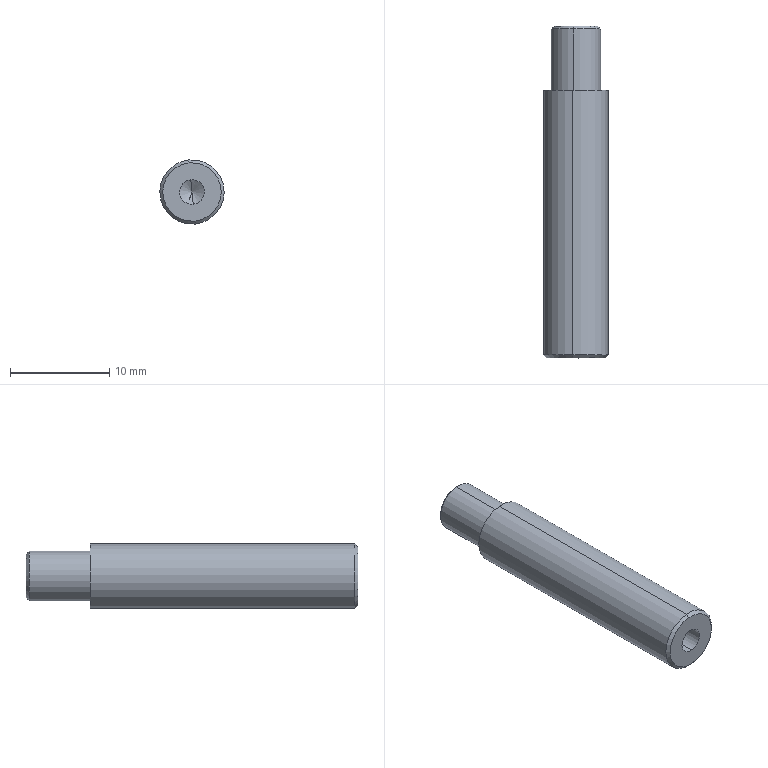Component | SolidWorks | DZ.KX.203-TC1505-30-09-01-05-12-1 | 1 solid | 15 faces | box 6.5 x 33.5 x 6.5 mm | volume 952 mm3 | cone 6 | cylinder 6 | plane 3 | commonest cylinder face diameters 2.5 x2 5 x2 6.5 x2 | material Plain Carbon Steel
build123d program:
from build123d import *

# Parameters (mm, degrees)
SKETCH1_R             = 3.25
BOSS_EXTRUDE1_DEPTH   = 27
SKETCH2_R             = 2.5
BOSS_EXTRUDE2_DEPTH   = 6.5
M3_TAPPED_HOLE1_D     = 2.5
M3_TAPPED_HOLE1_DEPTH = 14
M3_TAPPED_HOLE1_TIP   = 0.7511
CHAMFER1_SIZE         = 0.3


with BuildPart() as part:
    # Sketch1 → Boss-Extrude1 (new body)
    with BuildSketch(Plane(origin=(0, 0, 0), x_dir=(0, 0, -1), z_dir=(1, 0, 0))):
        Circle(SKETCH1_R)
    extrude(amount=BOSS_EXTRUDE1_DEPTH)

    # Sketch2 → Boss-Extrude2 (add)
    with BuildSketch(Plane.ZY):
        with Locations(Location((0, 0, 0), (0, 0, 180))):
            Circle(SKETCH2_R)
    extrude(amount=BOSS_EXTRUDE2_DEPTH)

    # M3 Tapped Hole1
    with Locations(Plane(origin=(27, 0, 0), x_dir=(0, 0, -1), z_dir=(1, 0, 0))):
        with Locations((0, 0)):
            Hole(M3_TAPPED_HOLE1_D / 2, depth=M3_TAPPED_HOLE1_DEPTH)
            with Locations((0, 0, -(M3_TAPPED_HOLE1_DEPTH + M3_TAPPED_HOLE1_TIP / 2))):  # 118° drill point
                Cone(0, M3_TAPPED_HOLE1_D / 2, M3_TAPPED_HOLE1_TIP, mode=Mode.SUBTRACT)

    # Chamfer1
    chamfer1_edges = [part.edges().sort_by_distance(p)[0] for p in [
        (27, 0, 3.25),
        (-6.5, 0, 2.5),
    ]]
    chamfer(chamfer1_edges, length=CHAMFER1_SIZE)


solid = part.part

# Placed as in the assembly
solid = solid.moved(Location((273.5, -525.807, -37.44), (0, 0, -90)))
STEP:
#1=COLOUR_RGB('',0.7922,0.8196,0.9333);
#2=FILL_AREA_STYLE_COLOUR('',#1);
#3=FILL_AREA_STYLE('',(#2));
#4=SURFACE_STYLE_FILL_AREA(#3);
#5=SURFACE_SIDE_STYLE('',(#4));
#6=SURFACE_STYLE_USAGE(.BOTH.,#5);
#7=PRESENTATION_STYLE_ASSIGNMENT((#6));
#8=CARTESIAN_POINT('',(10.759,-20.445,-1.388));
#9=VERTEX_POINT('',#8);
#10=CARTESIAN_POINT('',(10.776,-20.445,-1.56));
#11=VERTEX_POINT('',#10);
#12=CARTESIAN_POINT('',(10.768,-20.445,-1.474));
#13=DIRECTION('',(0.,1.,-0.));
#14=DIRECTION('',(-0.0993,0.,0.9951));
#15=AXIS2_PLACEMENT_3D('',#12,#13,#14);
#16=CIRCLE('',#15,0.08661);
#17=EDGE_CURVE('',#9,#11,#16,.T.);
#18=ORIENTED_EDGE('',*,*,#17,.F.);
#19=CARTESIAN_POINT('',(10.758,-20.457,-1.376));
#20=VERTEX_POINT('',#19);
#21=CARTESIAN_POINT('',(10.759,-20.445,-1.388));
#22=DIRECTION('',(-0.07022,-0.7071,0.7036));
#23=VECTOR('',#22,39.37);
#24=LINE('',#21,#23);
#25=EDGE_CURVE('',#9,#20,#24,.T.);
#26=ORIENTED_EDGE('',*,*,#25,.T.);
#27=CARTESIAN_POINT('',(10.777,-20.457,-1.572));
#28=VERTEX_POINT('',#27);
#29=CARTESIAN_POINT('',(10.768,-20.457,-1.474));
#30=DIRECTION('',(-0.,-1.,0.));
#31=DIRECTION('',(-0.0993,0.,0.9951));
#32=AXIS2_PLACEMENT_3D('',#29,#30,#31);
#33=CIRCLE('',#32,0.09843);
#34=EDGE_CURVE('',#28,#20,#33,.T.);
#35=ORIENTED_EDGE('',*,*,#34,.F.);
#36=CARTESIAN_POINT('',(10.776,-20.445,-1.56));
#37=DIRECTION('',(0.07022,-0.7071,-0.7036));
#38=VECTOR('',#37,39.37);
#39=LINE('',#36,#38);
#40=EDGE_CURVE('',#11,#28,#39,.T.);
#41=ORIENTED_EDGE('',*,*,#40,.F.);
#42=EDGE_LOOP('',(#18,#26,#35,#41));
#43=FACE_OUTER_BOUND('',#42,.T.);
#44=CARTESIAN_POINT('',(10.768,-20.445,-1.474));
#45=DIRECTION('',(-0.,-1.,0.));
#46=DIRECTION('',(0.0993,0.,-0.9951));
#47=AXIS2_PLACEMENT_3D('',#44,#45,#46);
#48=CONICAL_SURFACE('',#47,0.08661,0.7854);
#49=ADVANCED_FACE('',(#43),#48,.T.);
#50=CARTESIAN_POINT('',(10.779,-21.764,-1.59));
#51=VERTEX_POINT('',#50);
#52=CARTESIAN_POINT('',(10.756,-21.764,-1.358));
#53=VERTEX_POINT('',#52);
#54=CARTESIAN_POINT('',(10.768,-21.764,-1.474));
#55=DIRECTION('',(-0.,-1.,0.));
#56=DIRECTION('',(0.0993,0.,-0.9951));
#57=AXIS2_PLACEMENT_3D('',#54,#55,#56);
#58=CIRCLE('',#57,0.1161);
#59=EDGE_CURVE('',#51,#53,#58,.T.);
#60=ORIENTED_EDGE('',*,*,#59,.F.);
#61=CARTESIAN_POINT('',(10.78,-21.752,-1.601));
#62=VERTEX_POINT('',#61);
#63=CARTESIAN_POINT('',(10.779,-21.764,-1.59));
#64=DIRECTION('',(0.07022,0.7071,-0.7036));
#65=VECTOR('',#64,39.37);
#66=LINE('',#63,#65);
#67=EDGE_CURVE('',#51,#62,#66,.T.);
#68=ORIENTED_EDGE('',*,*,#67,.T.);
#69=CARTESIAN_POINT('',(10.755,-21.752,-1.347));
#70=VERTEX_POINT('',#69);
#71=CARTESIAN_POINT('',(10.768,-21.752,-1.474));
#72=DIRECTION('',(0.,1.,-0.));
#73=DIRECTION('',(0.0993,0.,-0.9951));
#74=AXIS2_PLACEMENT_3D('',#71,#72,#73);
#75=CIRCLE('',#74,0.128);
#76=EDGE_CURVE('',#70,#62,#75,.T.);
#77=ORIENTED_EDGE('',*,*,#76,.F.);
#78=CARTESIAN_POINT('',(10.756,-21.764,-1.358));
#79=DIRECTION('',(-0.07022,0.7071,0.7036));
#80=VECTOR('',#79,39.37);
#81=LINE('',#78,#80);
#82=EDGE_CURVE('',#53,#70,#81,.T.);
#83=ORIENTED_EDGE('',*,*,#82,.F.);
#84=EDGE_LOOP('',(#60,#68,#77,#83));
#85=FACE_OUTER_BOUND('',#84,.T.);
#86=CARTESIAN_POINT('',(10.768,-21.764,-1.474));
#87=DIRECTION('',(0.,1.,-0.));
#88=DIRECTION('',(-0.0993,0.,0.9951));
#89=AXIS2_PLACEMENT_3D('',#86,#87,#88);
#90=CONICAL_SURFACE('',#89,0.1161,0.7854);
#91=ADVANCED_FACE('',(#85),#90,.T.);
#92=CARTESIAN_POINT('',(10.763,-21.213,-1.425));
#93=VERTEX_POINT('',#92);
#94=CARTESIAN_POINT('',(10.773,-21.213,-1.523));
#95=VERTEX_POINT('',#94);
#96=CARTESIAN_POINT('',(10.768,-21.213,-1.474));
#97=DIRECTION('',(-0.,-1.,0.));
#98=DIRECTION('',(0.0993,0.,-0.9951));
#99=AXIS2_PLACEMENT_3D('',#96,#97,#98);
#100=CIRCLE('',#99,0.04921);
#101=EDGE_CURVE('',#93,#95,#100,.T.);
#102=ORIENTED_EDGE('',*,*,#101,.F.);
#103=CARTESIAN_POINT('',(10.763,-21.764,-1.425));
#104=VERTEX_POINT('',#103);
#105=CARTESIAN_POINT('',(10.763,-21.764,-1.425));
#106=DIRECTION('',(-0.,-1.,0.));
#107=VECTOR('',#106,39.37);
#108=LINE('',#105,#107);
#109=EDGE_CURVE('',#93,#104,#108,.T.);
#110=ORIENTED_EDGE('',*,*,#109,.T.);
#111=CARTESIAN_POINT('',(10.773,-21.764,-1.523));
#112=VERTEX_POINT('',#111);
#113=CARTESIAN_POINT('',(10.768,-21.764,-1.474));
#114=DIRECTION('',(-0.,-1.,0.));
#115=DIRECTION('',(0.0993,0.,-0.9951));
#116=AXIS2_PLACEMENT_3D('',#113,#114,#115);
#117=CIRCLE('',#116,0.04921);
#118=EDGE_CURVE('',#104,#112,#117,.T.);
#119=ORIENTED_EDGE('',*,*,#118,.T.);
#120=CARTESIAN_POINT('',(10.773,-21.764,-1.523));
#121=DIRECTION('',(-0.,-1.,0.));
#122=VECTOR('',#121,39.37);
#123=LINE('',#120,#122);
#124=EDGE_CURVE('',#95,#112,#123,.T.);
#125=ORIENTED_EDGE('',*,*,#124,.F.);
#126=EDGE_LOOP('',(#102,#110,#119,#125));
#127=FACE_OUTER_BOUND('',#126,.T.);
#128=CARTESIAN_POINT('',(10.768,-21.764,-1.474));
#129=DIRECTION('',(-0.,-1.,0.));
#130=DIRECTION('',(0.0993,0.,-0.9951));
#131=AXIS2_PLACEMENT_3D('',#128,#129,#130);
#132=CYLINDRICAL_SURFACE('',#131,0.04921);
#133=ADVANCED_FACE('',(#127),#132,.F.);
#134=CARTESIAN_POINT('',(10.768,-21.183,-1.474));
#135=VERTEX_POINT('',#134);
#136=CARTESIAN_POINT('',(10.773,-21.213,-1.523));
#137=DIRECTION('',(0.08512,-0.515,-0.8529));
#138=VECTOR('',#137,39.37);
#139=LINE('',#136,#138);
#140=EDGE_CURVE('',#135,#95,#139,.T.);
#141=ORIENTED_EDGE('',*,*,#140,.F.);
#142=CARTESIAN_POINT('',(10.763,-21.213,-1.425));
#143=DIRECTION('',(-0.08512,-0.515,0.8529));
#144=VECTOR('',#143,39.37);
#145=LINE('',#142,#144);
#146=EDGE_CURVE('',#135,#93,#145,.T.);
#147=ORIENTED_EDGE('',*,*,#146,.T.);
#148=ORIENTED_EDGE('',*,*,#101,.T.);
#149=EDGE_LOOP('',(#141,#147,#148));
#150=FACE_OUTER_BOUND('',#149,.T.);
#151=CARTESIAN_POINT('',(10.768,-21.213,-1.474));
#152=DIRECTION('',(-0.,-1.,0.));
#153=DIRECTION('',(0.0993,0.,-0.9951));
#154=AXIS2_PLACEMENT_3D('',#151,#152,#153);
#155=CONICAL_SURFACE('',#154,0.04921,1.03);
#156=ADVANCED_FACE('',(#150),#155,.F.);
#157=ORIENTED_EDGE('',*,*,#34,.T.);
#158=CARTESIAN_POINT('',(10.758,-20.701,-1.376));
#159=VERTEX_POINT('',#158);
#160=CARTESIAN_POINT('',(10.758,-20.445,-1.376));
#161=DIRECTION('',(-0.,-1.,0.));
#162=VECTOR('',#161,39.37);
#163=LINE('',#160,#162);
#164=EDGE_CURVE('',#20,#159,#163,.T.);
#165=ORIENTED_EDGE('',*,*,#164,.T.);
#166=CARTESIAN_POINT('',(10.777,-20.701,-1.572));
#167=VERTEX_POINT('',#166);
#168=CARTESIAN_POINT('',(10.768,-20.701,-1.474));
#169=DIRECTION('',(0.,1.,-0.));
#170=DIRECTION('',(0.0993,0.,-0.9951));
#171=AXIS2_PLACEMENT_3D('',#168,#169,#170);
#172=CIRCLE('',#171,0.09843);
#173=EDGE_CURVE('',#159,#167,#172,.T.);
#174=ORIENTED_EDGE('',*,*,#173,.T.);
#175=CARTESIAN_POINT('',(10.777,-20.445,-1.572));
#176=DIRECTION('',(-0.,-1.,0.));
#177=VECTOR('',#176,39.37);
#178=LINE('',#175,#177);
#179=EDGE_CURVE('',#28,#167,#178,.T.);
#180=ORIENTED_EDGE('',*,*,#179,.F.);
#181=EDGE_LOOP('',(#157,#165,#174,#180));
#182=FACE_OUTER_BOUND('',#181,.T.);
#183=CARTESIAN_POINT('',(10.768,-20.445,-1.474));
#184=DIRECTION('',(-0.,-1.,0.));
#185=DIRECTION('',(0.0993,0.,-0.9951));
#186=AXIS2_PLACEMENT_3D('',#183,#184,#185);
#187=CYLINDRICAL_SURFACE('',#186,0.09843);
#188=ADVANCED_FACE('',(#182),#187,.T.);
#189=ORIENTED_EDGE('',*,*,#76,.T.);
#190=CARTESIAN_POINT('',(10.78,-20.701,-1.601));
#191=VERTEX_POINT('',#190);
#192=CARTESIAN_POINT('',(10.78,-21.764,-1.601));
#193=DIRECTION('',(0.,1.,-0.));
#194=VECTOR('',#193,39.37);
#195=LINE('',#192,#194);
#196=EDGE_CURVE('',#62,#191,#195,.T.);
#197=ORIENTED_EDGE('',*,*,#196,.T.);
#198=CARTESIAN_POINT('',(10.755,-20.701,-1.347));
#199=VERTEX_POINT('',#198);
#200=CARTESIAN_POINT('',(10.768,-20.701,-1.474));
#201=DIRECTION('',(-0.,-1.,0.));
#202=DIRECTION('',(0.0993,0.,-0.9951));
#203=AXIS2_PLACEMENT_3D('',#200,#201,#202);
#204=CIRCLE('',#203,0.128);
#205=EDGE_CURVE('',#191,#199,#204,.T.);
#206=ORIENTED_EDGE('',*,*,#205,.T.);
#207=CARTESIAN_POINT('',(10.755,-21.764,-1.347));
#208=DIRECTION('',(0.,1.,-0.));
#209=VECTOR('',#208,39.37);
#210=LINE('',#207,#209);
#211=EDGE_CURVE('',#70,#199,#210,.T.);
#212=ORIENTED_EDGE('',*,*,#211,.F.);
#213=EDGE_LOOP('',(#189,#197,#206,#212));
#214=FACE_OUTER_BOUND('',#213,.T.);
#215=CARTESIAN_POINT('',(10.768,-21.764,-1.474));
#216=DIRECTION('',(0.,1.,-0.));
#217=DIRECTION('',(-0.0993,0.,0.9951));
#218=AXIS2_PLACEMENT_3D('',#215,#216,#217);
#219=CYLINDRICAL_SURFACE('',#218,0.128);
#220=ADVANCED_FACE('',(#214),#219,.T.);
#221=CARTESIAN_POINT('',(10.768,-20.701,-1.474));
#222=DIRECTION('',(-0.,-1.,0.));
#223=DIRECTION('',(0.0993,0.,-0.9951));
#224=AXIS2_PLACEMENT_3D('',#221,#222,#223);
#225=CIRCLE('',#224,0.128);
#226=EDGE_CURVE('',#199,#191,#225,.T.);
#227=ORIENTED_EDGE('',*,*,#226,.F.);
#228=ORIENTED_EDGE('',*,*,#205,.F.);
#229=EDGE_LOOP('',(#227,#228));
#230=FACE_OUTER_BOUND('',#229,.T.);
#231=CARTESIAN_POINT('',(10.768,-20.701,-1.474));
#232=DIRECTION('',(0.,1.,-0.));
#233=DIRECTION('',(0.0993,0.,-0.9951));
#234=AXIS2_PLACEMENT_3D('',#231,#232,#233);
#235=CIRCLE('',#234,0.09843);
#236=EDGE_CURVE('',#167,#159,#235,.T.);
#237=ORIENTED_EDGE('',*,*,#236,.F.);
#238=ORIENTED_EDGE('',*,*,#173,.F.);
#239=EDGE_LOOP('',(#237,#238));
#240=FACE_BOUND('',#239,.T.);
#241=CARTESIAN_POINT('',(10.768,-20.701,-1.474));
#242=DIRECTION('',(-0.,-1.,0.));
#243=DIRECTION('',(0.0993,-0.,-0.9951));
#244=AXIS2_PLACEMENT_3D('',#241,#242,#243);
#245=PLANE('',#244);
#246=ADVANCED_FACE('',(#230,#240),#245,.F.);
#247=ORIENTED_EDGE('',*,*,#196,.F.);
#248=CARTESIAN_POINT('',(10.768,-21.752,-1.474));
#249=DIRECTION('',(0.,1.,-0.));
#250=DIRECTION('',(0.0993,0.,-0.9951));
#251=AXIS2_PLACEMENT_3D('',#248,#249,#250);
#252=CIRCLE('',#251,0.128);
#253=EDGE_CURVE('',#62,#70,#252,.T.);
#254=ORIENTED_EDGE('',*,*,#253,.T.);
#255=ORIENTED_EDGE('',*,*,#211,.T.);
#256=ORIENTED_EDGE('',*,*,#226,.T.);
#257=EDGE_LOOP('',(#247,#254,#255,#256));
#258=FACE_OUTER_BOUND('',#257,.T.);
#259=CARTESIAN_POINT('',(10.768,-21.764,-1.474));
#260=DIRECTION('',(0.,1.,-0.));
#261=DIRECTION('',(-0.0993,0.,0.9951));
#262=AXIS2_PLACEMENT_3D('',#259,#260,#261);
#263=CYLINDRICAL_SURFACE('',#262,0.128);
#264=ADVANCED_FACE('',(#258),#263,.T.);
#265=CARTESIAN_POINT('',(10.768,-21.764,-1.474));
#266=DIRECTION('',(-0.,-1.,0.));
#267=DIRECTION('',(0.0993,0.,-0.9951));
#268=AXIS2_PLACEMENT_3D('',#265,#266,#267);
#269=CIRCLE('',#268,0.1161);
#270=EDGE_CURVE('',#53,#51,#269,.T.);
#271=ORIENTED_EDGE('',*,*,#270,.T.);
#272=ORIENTED_EDGE('',*,*,#59,.T.);
#273=EDGE_LOOP('',(#271,#272));
#274=FACE_OUTER_BOUND('',#273,.T.);
#275=CARTESIAN_POINT('',(10.768,-21.764,-1.474));
#276=DIRECTION('',(-0.,-1.,0.));
#277=DIRECTION('',(0.0993,0.,-0.9951));
#278=AXIS2_PLACEMENT_3D('',#275,#276,#277);
#279=CIRCLE('',#278,0.04921);
#280=EDGE_CURVE('',#112,#104,#279,.T.);
#281=ORIENTED_EDGE('',*,*,#280,.F.);
#282=ORIENTED_EDGE('',*,*,#118,.F.);
#283=EDGE_LOOP('',(#281,#282));
#284=FACE_BOUND('',#283,.T.);
#285=CARTESIAN_POINT('',(10.768,-21.764,-1.474));
#286=DIRECTION('',(-0.,-1.,0.));
#287=DIRECTION('',(0.0993,-0.,-0.9951));
#288=AXIS2_PLACEMENT_3D('',#285,#286,#287);
#289=PLANE('',#288);
#290=ADVANCED_FACE('',(#274,#284),#289,.T.);
#291=ORIENTED_EDGE('',*,*,#164,.F.);
#292=CARTESIAN_POINT('',(10.768,-20.457,-1.474));
#293=DIRECTION('',(-0.,-1.,0.));
#294=DIRECTION('',(-0.0993,0.,0.9951));
#295=AXIS2_PLACEMENT_3D('',#292,#293,#294);
#296=CIRCLE('',#295,0.09843);
#297=EDGE_CURVE('',#20,#28,#296,.T.);
#298=ORIENTED_EDGE('',*,*,#297,.T.);
#299=ORIENTED_EDGE('',*,*,#179,.T.);
#300=ORIENTED_EDGE('',*,*,#236,.T.);
#301=EDGE_LOOP('',(#291,#298,#299,#300));
#302=FACE_OUTER_BOUND('',#301,.T.);
#303=CARTESIAN_POINT('',(10.768,-20.445,-1.474));
#304=DIRECTION('',(-0.,-1.,0.));
#305=DIRECTION('',(0.0993,0.,-0.9951));
#306=AXIS2_PLACEMENT_3D('',#303,#304,#305);
#307=CYLINDRICAL_SURFACE('',#306,0.09843);
#308=ADVANCED_FACE('',(#302),#307,.T.);
#309=CARTESIAN_POINT('',(10.768,-20.445,-1.474));
#310=DIRECTION('',(0.,1.,-0.));
#311=DIRECTION('',(-0.0993,0.,0.9951));
#312=AXIS2_PLACEMENT_3D('',#309,#310,#311);
#313=CIRCLE('',#312,0.08661);
#314=EDGE_CURVE('',#11,#9,#313,.T.);
#315=ORIENTED_EDGE('',*,*,#314,.T.);
#316=ORIENTED_EDGE('',*,*,#17,.T.);
#317=EDGE_LOOP('',(#315,#316));
#318=FACE_OUTER_BOUND('',#317,.T.);
#319=CARTESIAN_POINT('',(10.768,-20.445,-1.474));
#320=DIRECTION('',(0.,1.,-0.));
#321=DIRECTION('',(-0.0993,0.,0.9951));
#322=AXIS2_PLACEMENT_3D('',#319,#320,#321);
#323=PLANE('',#322);
#324=ADVANCED_FACE('',(#318),#323,.T.);
#325=ORIENTED_EDGE('',*,*,#146,.F.);
#326=ORIENTED_EDGE('',*,*,#140,.T.);
#327=CARTESIAN_POINT('',(10.768,-21.213,-1.474));
#328=DIRECTION('',(-0.,-1.,0.));
#329=DIRECTION('',(0.0993,0.,-0.9951));
#330=AXIS2_PLACEMENT_3D('',#327,#328,#329);
#331=CIRCLE('',#330,0.04921);
#332=EDGE_CURVE('',#95,#93,#331,.T.);
#333=ORIENTED_EDGE('',*,*,#332,.T.);
#334=EDGE_LOOP('',(#325,#326,#333));
#335=FACE_OUTER_BOUND('',#334,.T.);
#336=CARTESIAN_POINT('',(10.768,-21.213,-1.474));
#337=DIRECTION('',(-0.,-1.,0.));
#338=DIRECTION('',(0.0993,0.,-0.9951));
#339=AXIS2_PLACEMENT_3D('',#336,#337,#338);
#340=CONICAL_SURFACE('',#339,0.04921,1.03);
#341=ADVANCED_FACE('',(#335),#340,.F.);
#342=ORIENTED_EDGE('',*,*,#109,.F.);
#343=ORIENTED_EDGE('',*,*,#332,.F.);
#344=ORIENTED_EDGE('',*,*,#124,.T.);
#345=ORIENTED_EDGE('',*,*,#280,.T.);
#346=EDGE_LOOP('',(#342,#343,#344,#345));
#347=FACE_OUTER_BOUND('',#346,.T.);
#348=CARTESIAN_POINT('',(10.768,-21.764,-1.474));
#349=DIRECTION('',(-0.,-1.,0.));
#350=DIRECTION('',(0.0993,0.,-0.9951));
#351=AXIS2_PLACEMENT_3D('',#348,#349,#350);
#352=CYLINDRICAL_SURFACE('',#351,0.04921);
#353=ADVANCED_FACE('',(#347),#352,.F.);
#354=ORIENTED_EDGE('',*,*,#67,.F.);
#355=ORIENTED_EDGE('',*,*,#270,.F.);
#356=ORIENTED_EDGE('',*,*,#82,.T.);
#357=ORIENTED_EDGE('',*,*,#253,.F.);
#358=EDGE_LOOP('',(#354,#355,#356,#357));
#359=FACE_OUTER_BOUND('',#358,.T.);
#360=CARTESIAN_POINT('',(10.768,-21.764,-1.474));
#361=DIRECTION('',(0.,1.,-0.));
#362=DIRECTION('',(-0.0993,0.,0.9951));
#363=AXIS2_PLACEMENT_3D('',#360,#361,#362);
#364=CONICAL_SURFACE('',#363,0.1161,0.7854);
#365=ADVANCED_FACE('',(#359),#364,.T.);
#366=ORIENTED_EDGE('',*,*,#25,.F.);
#367=ORIENTED_EDGE('',*,*,#314,.F.);
#368=ORIENTED_EDGE('',*,*,#40,.T.);
#369=ORIENTED_EDGE('',*,*,#297,.F.);
#370=EDGE_LOOP('',(#366,#367,#368,#369));
#371=FACE_OUTER_BOUND('',#370,.T.);
#372=CARTESIAN_POINT('',(10.768,-20.445,-1.474));
#373=DIRECTION('',(-0.,-1.,0.));
#374=DIRECTION('',(0.0993,0.,-0.9951));
#375=AXIS2_PLACEMENT_3D('',#372,#373,#374);
#376=CONICAL_SURFACE('',#375,0.08661,0.7854);
#377=ADVANCED_FACE('',(#371),#376,.T.);
#378=CLOSED_SHELL('',(#49,#91,#133,#156,#188,#220,#246,#264,#290,#308,#324,#341,#353,#365,#377));
#379=MANIFOLD_SOLID_BREP('',#378);
#380=STYLED_ITEM('',(#7),#379);
#381=(LENGTH_UNIT()NAMED_UNIT(*)SI_UNIT($,.METRE.));
#382=LENGTH_MEASURE_WITH_UNIT(LENGTH_MEASURE(0.0254),#381);
#383=DIMENSIONAL_EXPONENTS(1.,0.,0.,0.,0.,0.,0.);
#384=(CONVERSION_BASED_UNIT('',#382)LENGTH_UNIT()NAMED_UNIT(#383));
#385=UNCERTAINTY_MEASURE_WITH_UNIT(LENGTH_MEASURE(0.00001),#384,'','');
#386=(NAMED_UNIT(*)PLANE_ANGLE_UNIT()SI_UNIT($,.RADIAN.));
#387=(NAMED_UNIT(*)SI_UNIT($,.STERADIAN.)SOLID_ANGLE_UNIT());
#388=(GEOMETRIC_REPRESENTATION_CONTEXT(3)GLOBAL_UNCERTAINTY_ASSIGNED_CONTEXT((#385))GLOBAL_UNIT_ASSIGNED_CONTEXT((#384,#386,#387))REPRESENTATION_CONTEXT('',''));
#389=MECHANICAL_DESIGN_GEOMETRIC_PRESENTATION_REPRESENTATION('',(#380),#388);
#390=PRESENTATION_LAYER_ASSIGNMENT('','',(#380));
#391=CARTESIAN_POINT('',(0.,0.,0.));
#392=DIRECTION('',(0.,0.,1.));
#393=DIRECTION('',(1.,0.,0.));
#394=AXIS2_PLACEMENT_3D('',#391,#392,#393);
#395=(LENGTH_UNIT()NAMED_UNIT(*)SI_UNIT($,.METRE.));
#396=LENGTH_MEASURE_WITH_UNIT(LENGTH_MEASURE(0.0254),#395);
#397=DIMENSIONAL_EXPONENTS(1.,0.,0.,0.,0.,0.,0.);
#398=(CONVERSION_BASED_UNIT('',#396)LENGTH_UNIT()NAMED_UNIT(#397));
#399=UNCERTAINTY_MEASURE_WITH_UNIT(LENGTH_MEASURE(0.00001),#398,'','');
#400=(NAMED_UNIT(*)PLANE_ANGLE_UNIT()SI_UNIT($,.RADIAN.));
#401=(NAMED_UNIT(*)SI_UNIT($,.STERADIAN.)SOLID_ANGLE_UNIT());
#402=(GEOMETRIC_REPRESENTATION_CONTEXT(3)GLOBAL_UNCERTAINTY_ASSIGNED_CONTEXT((#399))GLOBAL_UNIT_ASSIGNED_CONTEXT((#398,#400,#401))REPRESENTATION_CONTEXT('',''));
#403=ADVANCED_BREP_SHAPE_REPRESENTATION('',(#379,#394),#402);